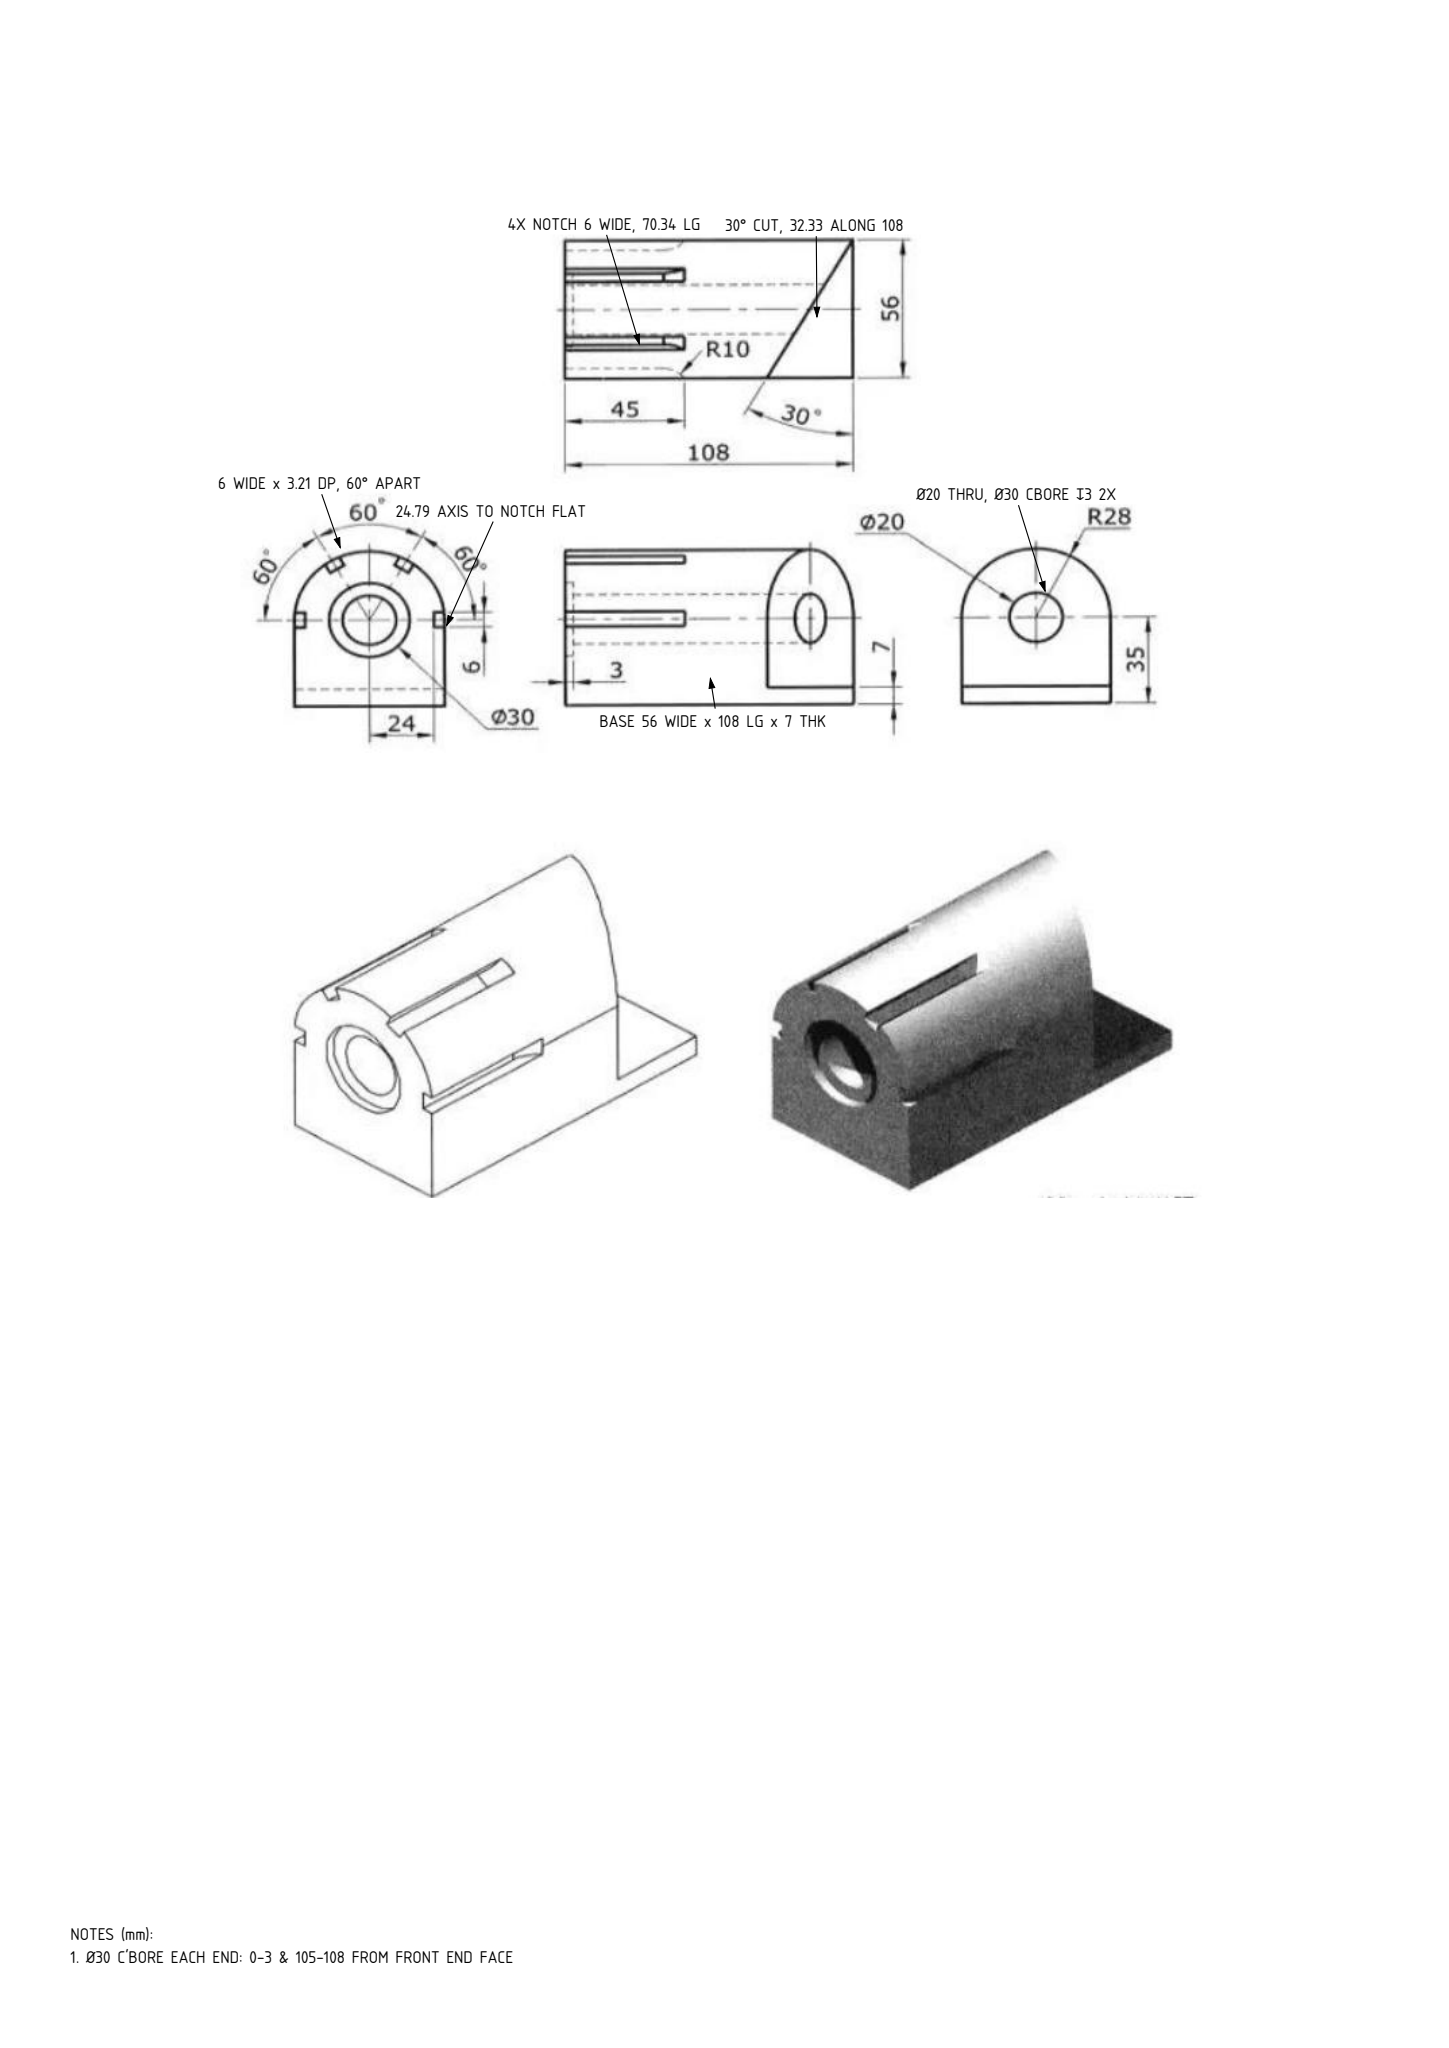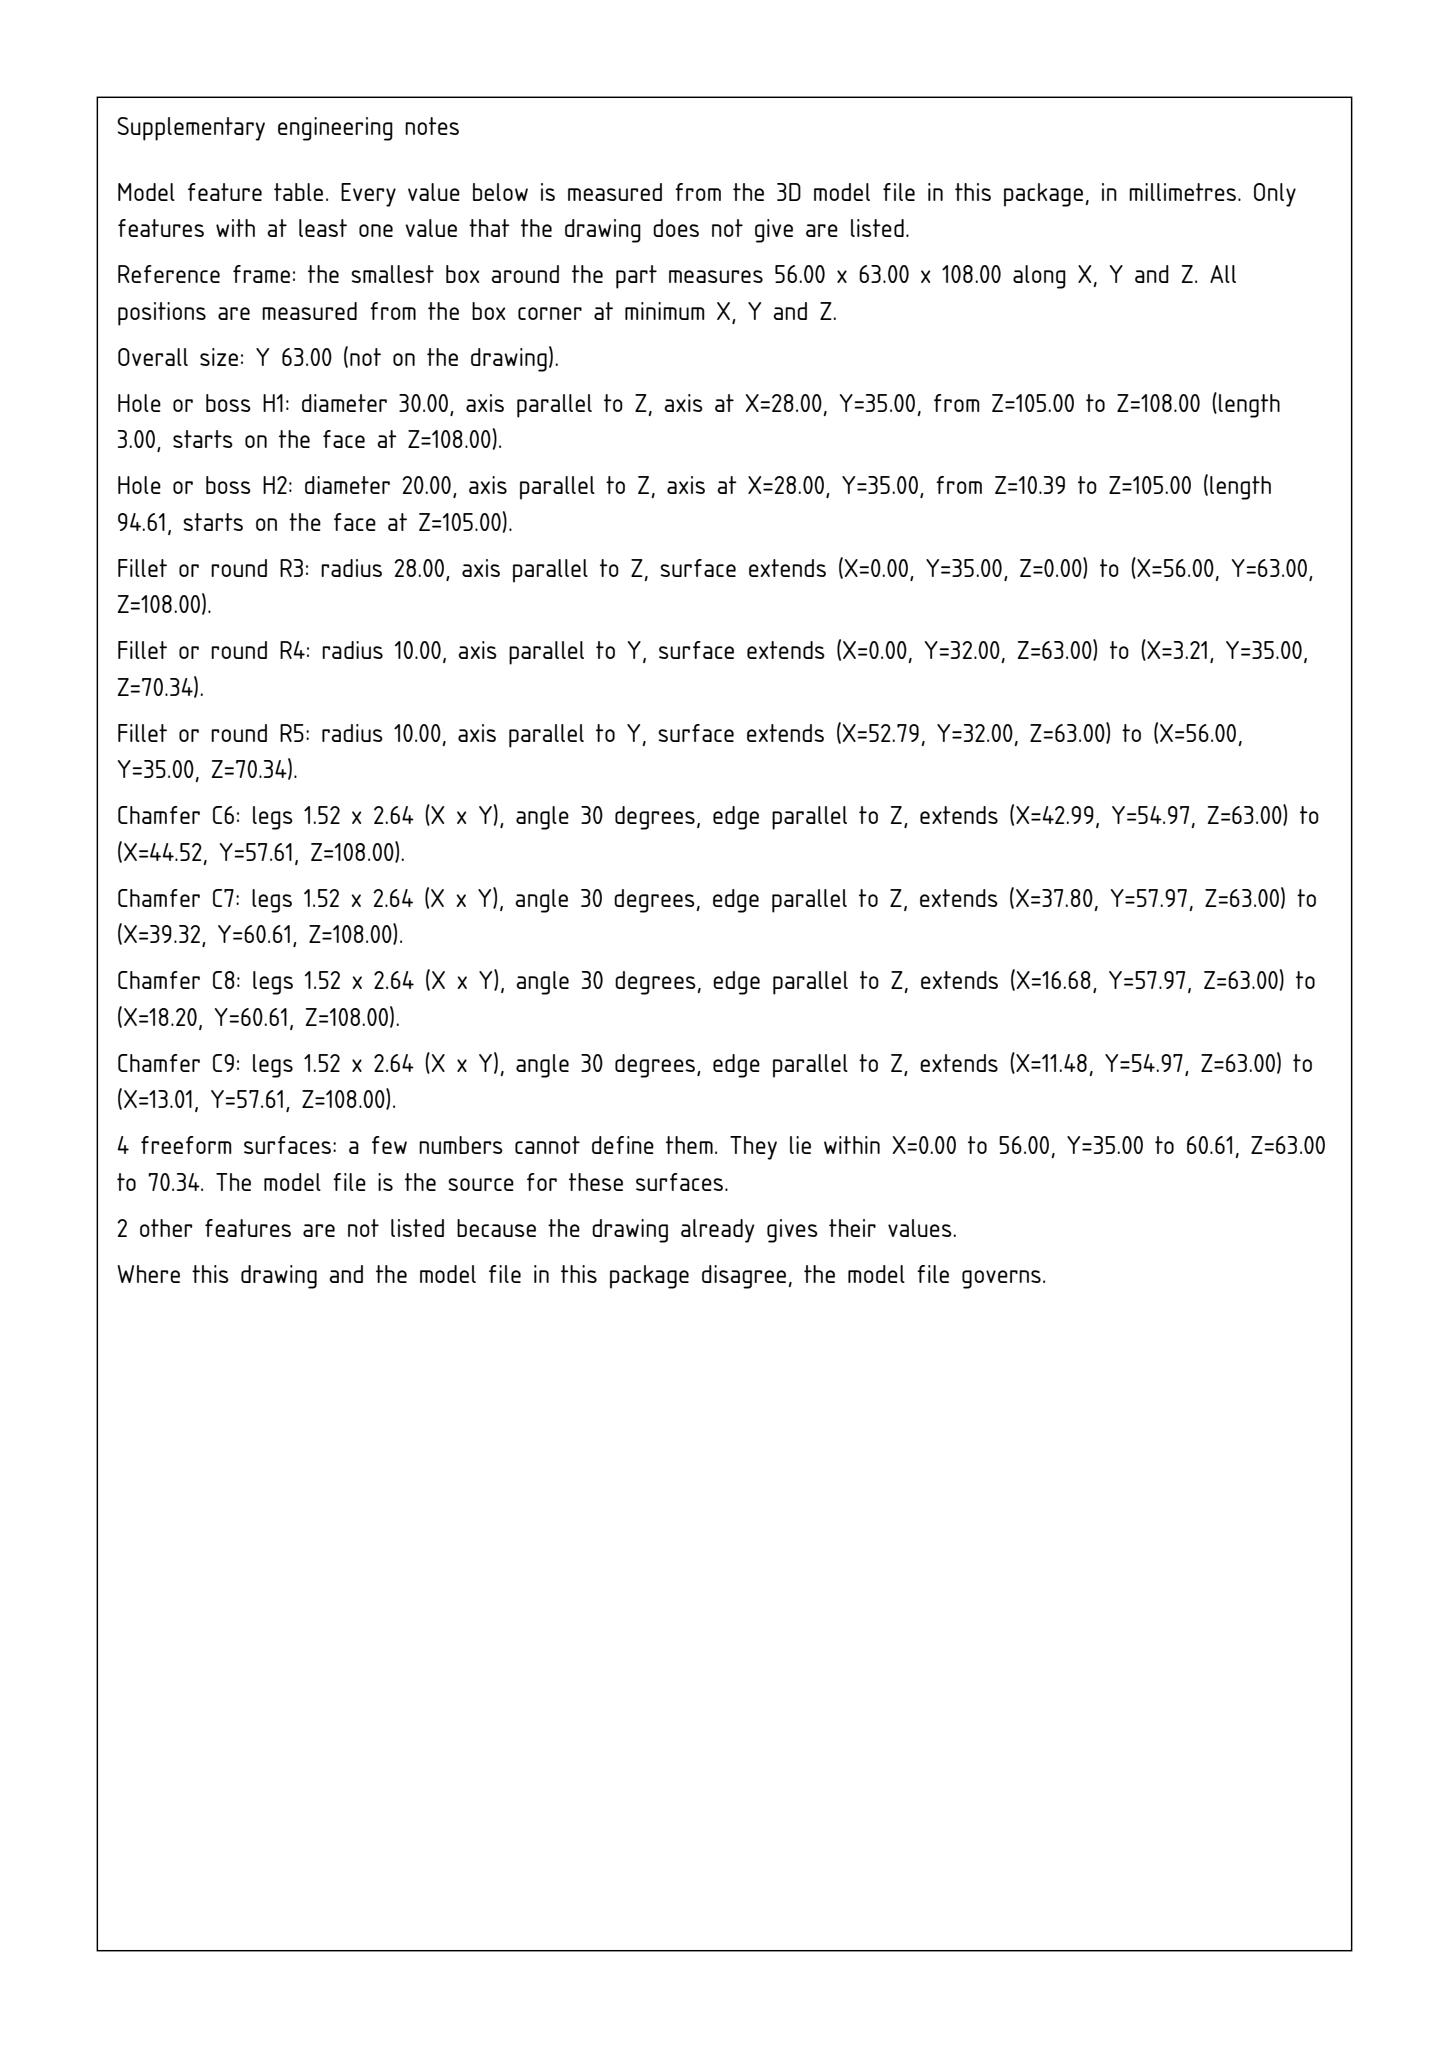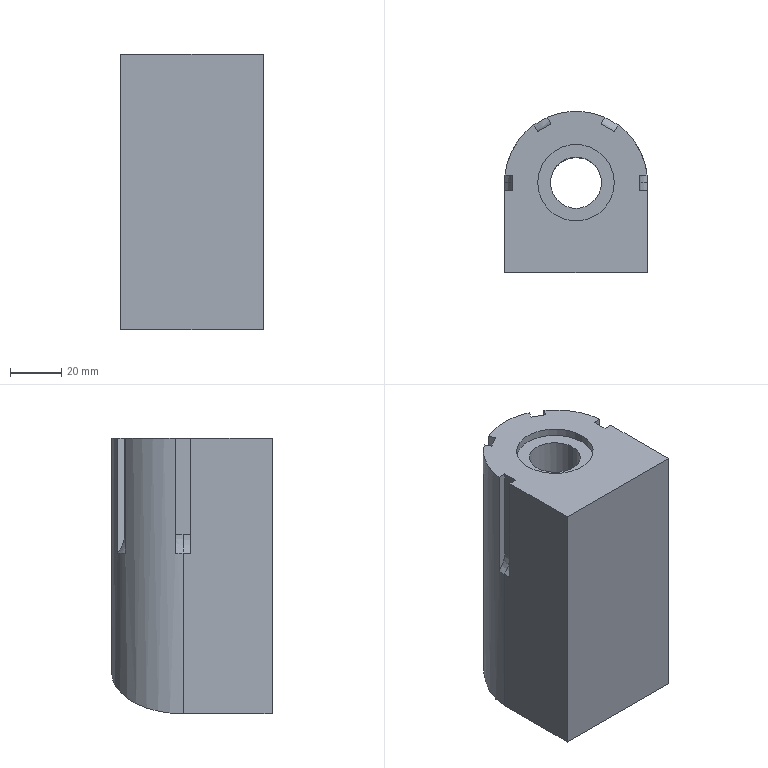Part | SolidWorks | mm | 1 solid | 31 faces | box 56 x 63 x 108 mm | volume 266152 mm3 | plane 20 | cylinder 7 | spline 4 | commonest cylinder face diameters 20 x4 30 x2 56 x1
Drawing notes:
Ø20 THRU, Ø30 C'BORE DP 3 BOTH ENDS | from the solid: Ø30 z-cylinders at (28,35) len 3.0, count 2; Ø20 z-bore at (28,35)
NOTCHES ON Ø56 OD: 6 WIDE x 3.21 DEEP (TO R24.79), 60° APART | from the solid: y-planes 32 & 38 (6 wide); x-planes 3.21 & 52.79 vs Ø56 OD ctr x=28 -> 3.21 deep
Ø30 C'BORE EACH END: 0-3 & 105-108 FROM FRONT END FACE | from the solid: z-planes 0, 105, 108; two Ø30 cyls len 3 at each end of 108 long Ø56 body
BASE PLATE 56 WIDE x 108 LG x 7 THK, FLUSH W/ Ø56 OD | from the solid: bbox_xyz x=56.001 (= Ø56 OD), z=108.001; y-plane at 7.0 = plate top; Ø56 cyl length 108
NOTCH 6 WIDE x 3.21 DP, 70.34 LG TO R10 RUNOUT - 4X 60° APART | from the solid: y-planes 32.0 & 38.0 (6 wide, ctr y=35); x-planes 3.21 & 52.79 = 28-24.79 (3.21 dp from Ø56 OD); Ø20 y-axis cutter cyls at z=70.34 (R10 runout; breakout at z=63 = 45 from z=108 end)
30° CUT RUNS 32.33 ALONG 108 FROM END CORNER; BORE 94.61 LG | from the solid: 56 x tan30 = 32.33 across full 56 width; Ø20 z-bore face length 94.61 = 105 - 10.39 (plane cuts bore 18/38 off-ctr)
24 REF = 24.79 FROM AXIS TO NOTCH FLAT (3.21 DP FROM Ø56 OD) | from the solid: Ø56 axis x=28; notch flats x-planes 3.21 & 52.79 -> 28-3.21 = 24.79 from axis